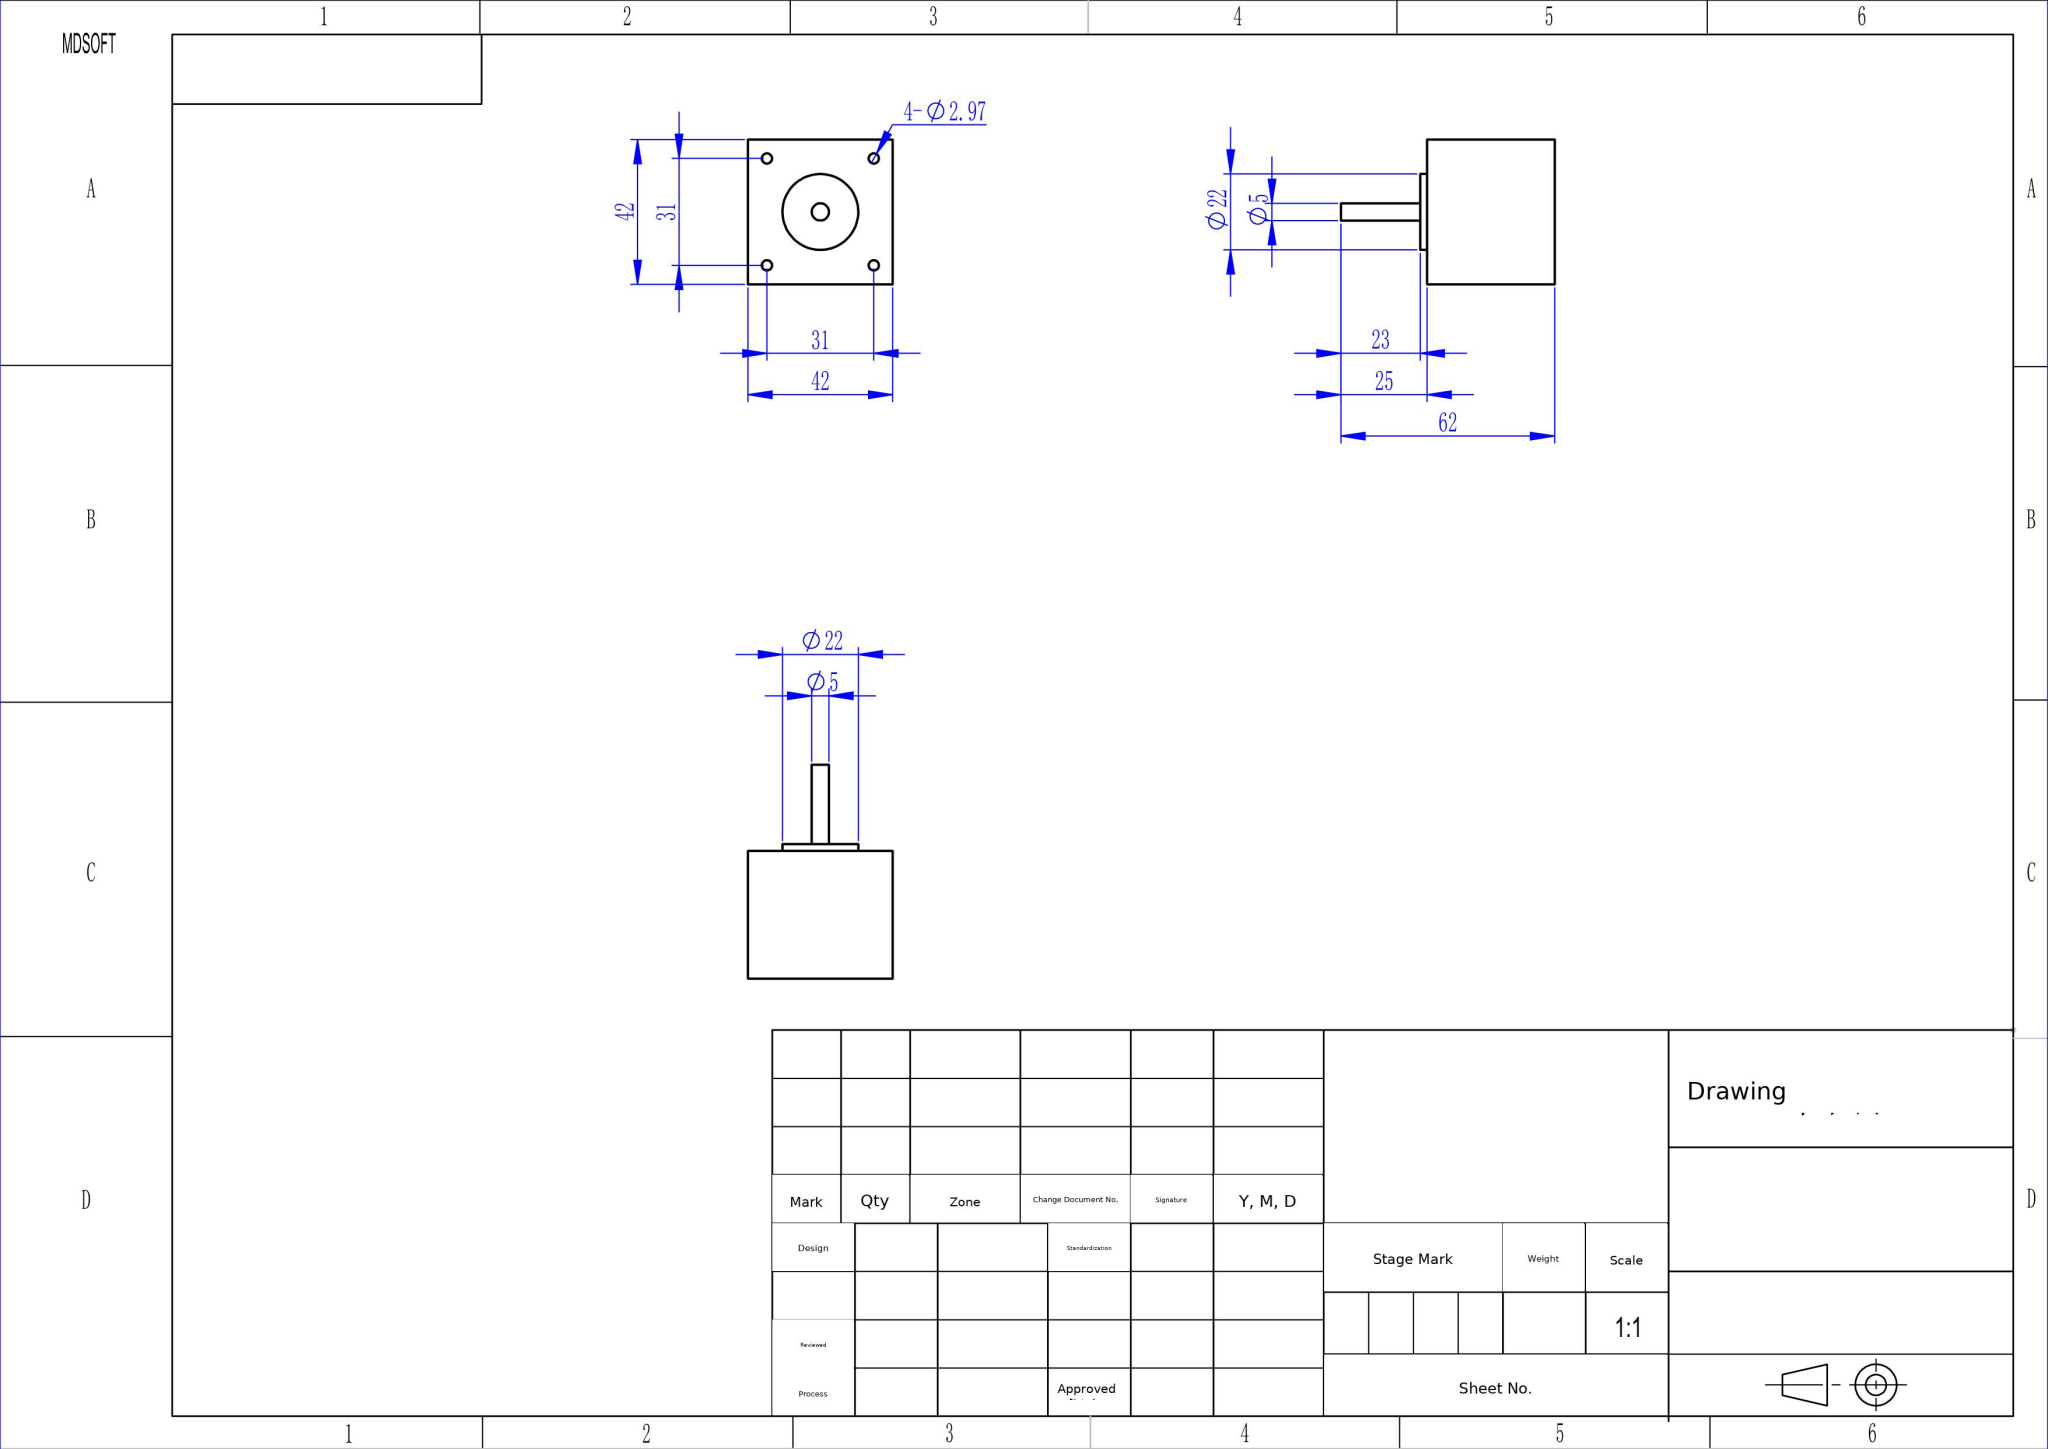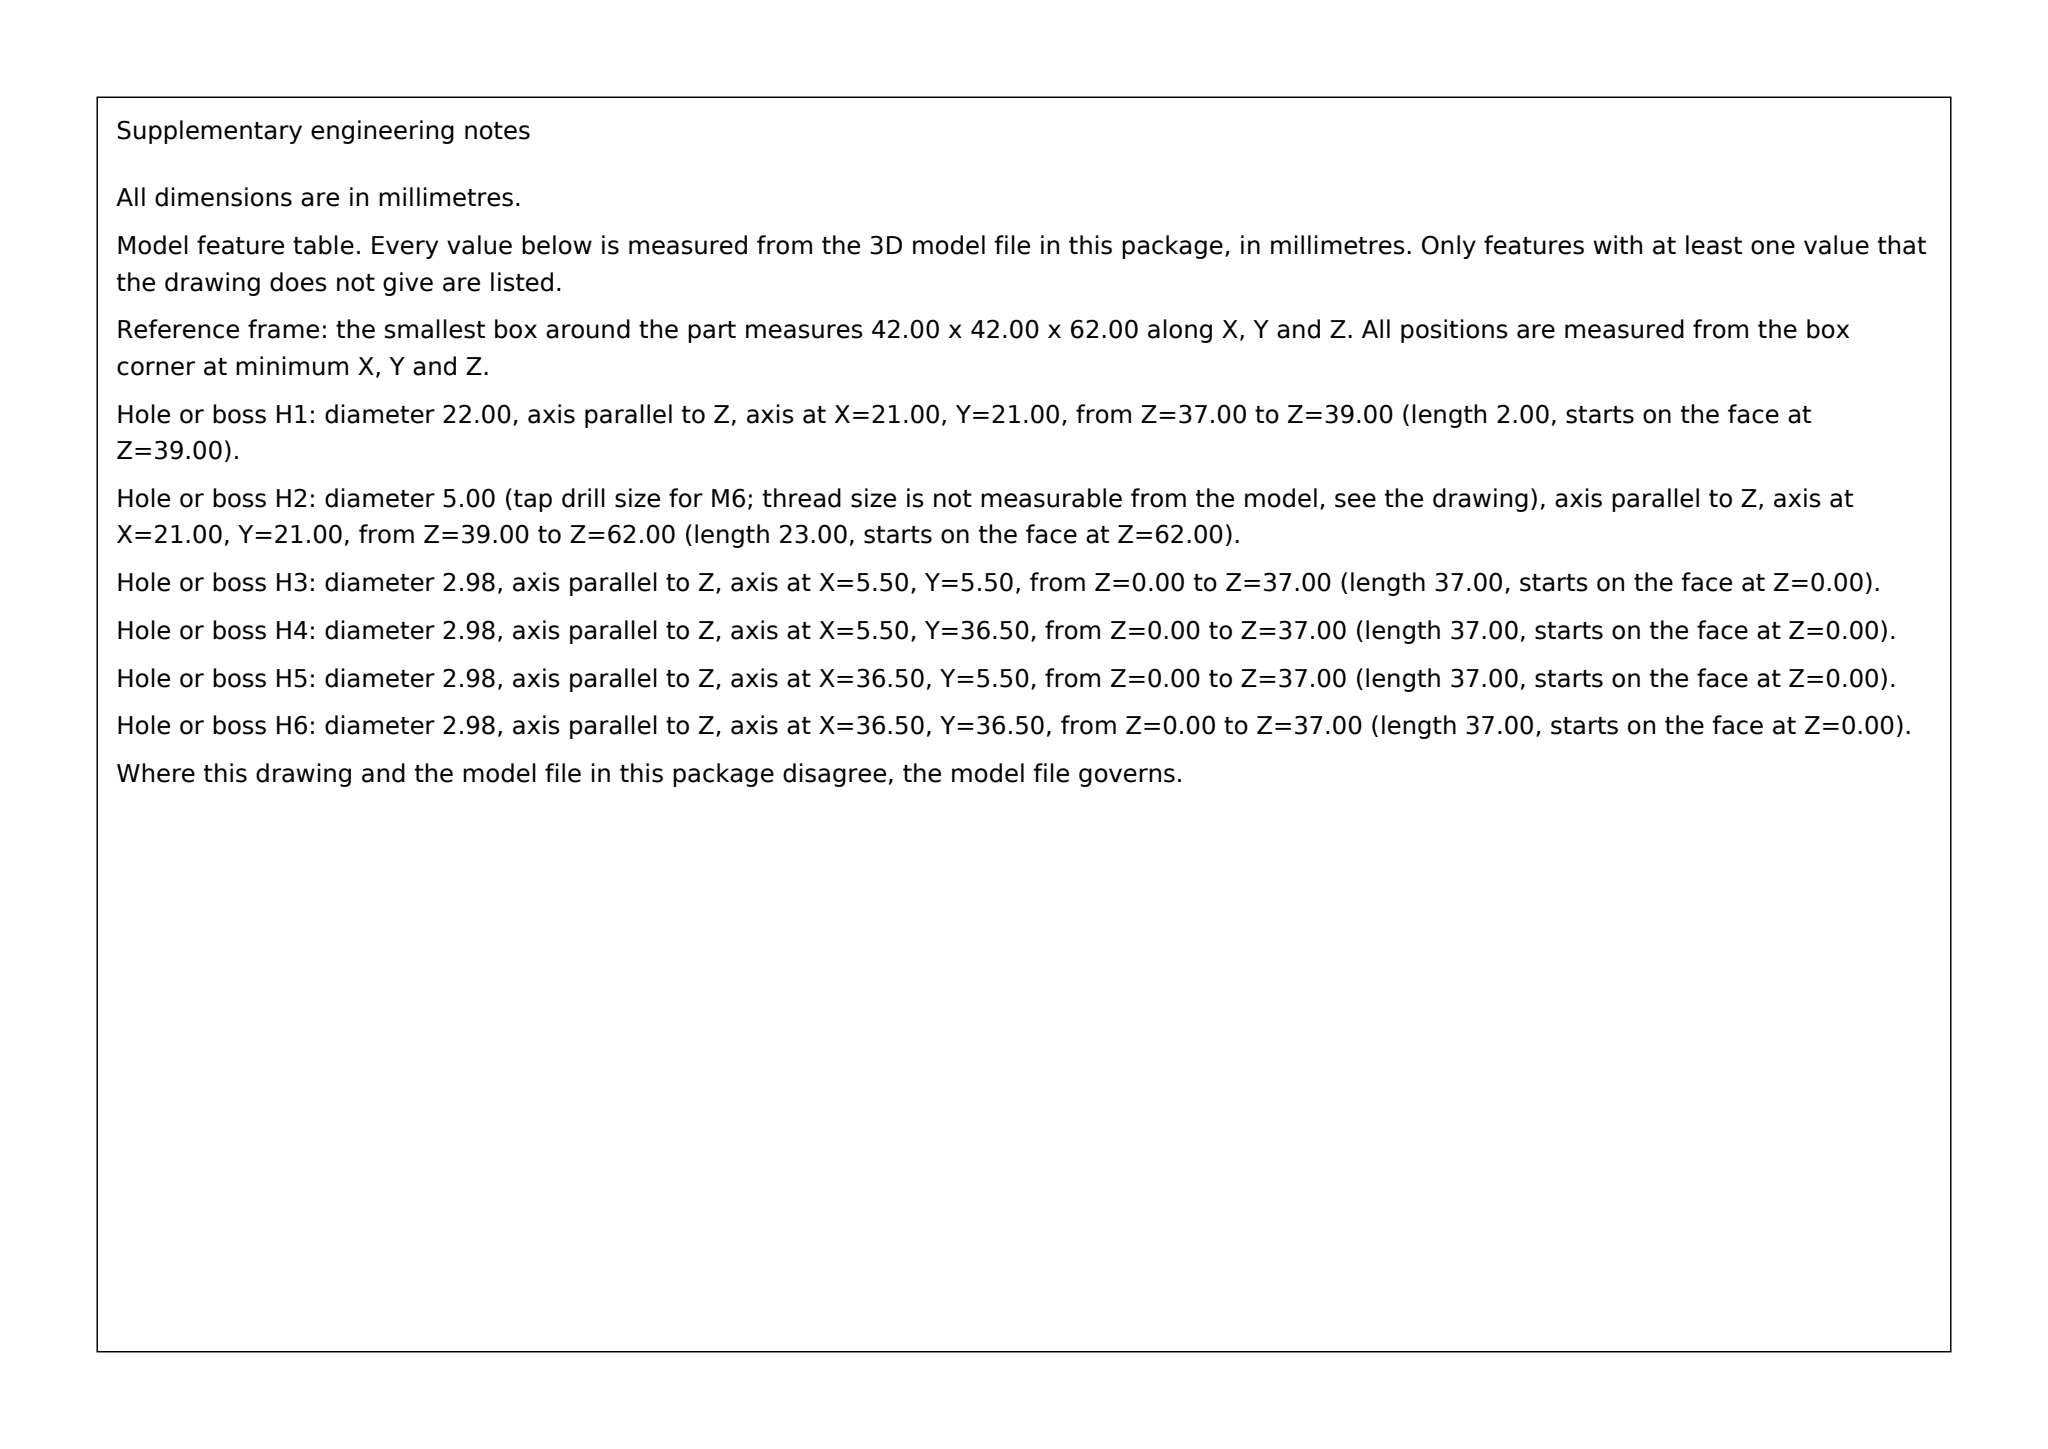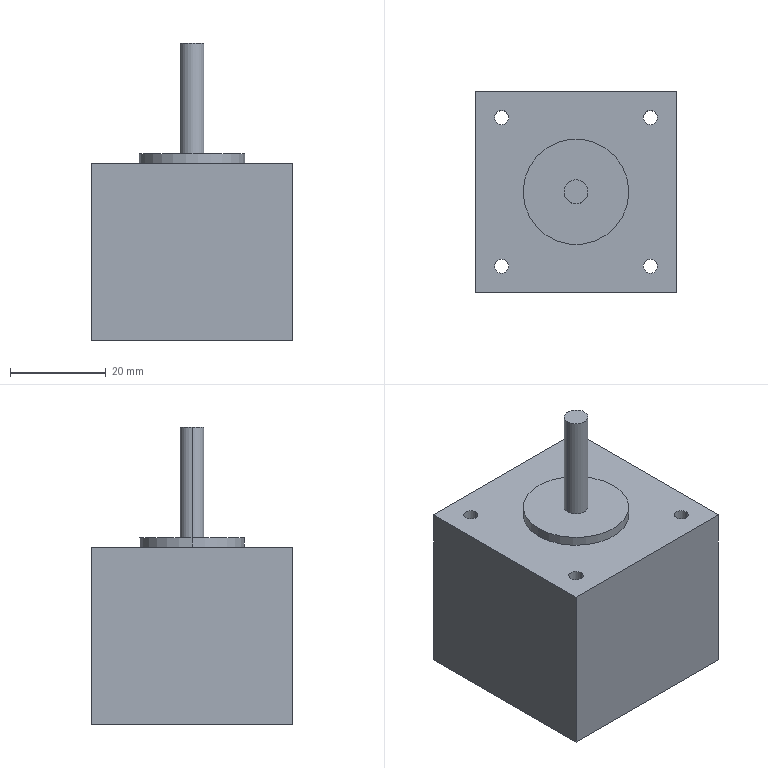Part | SolidWorks | mm | 1 solid | 20 faces | box 42 x 42 x 62 mm | volume 65453 mm3 | cylinder 12 | plane 8 | commonest cylinder face diameters 2.972 x8 5 x2 22 x2
build123d program:
from build123d import *

# Parameters (mm, degrees)
SKETCH1_W           = 42
SKETCH1_H           = 42
SKETCH1_R           = 1.486
BOSS_EXTRUDE1_DEPTH = 37
SKETCH3_3_R         = 2.5
BOSS_EXTRUDE2_DEPTH = 25
SKETCH3_3_2_R       = 11
SKETCH3_3_2_R_2     = 2.5
BOSS_EXTRUDE3_DEPTH = 2


with BuildPart() as part:
    # Sketch1 → Boss-Extrude1 (new body)
    with BuildSketch(Plane.XY):
        with Locations((-1.97, 1.739)):
            Rectangle(SKETCH1_W, SKETCH1_H)
        with Locations((-17.47, 17.239)):
            Circle(SKETCH1_R, mode=Mode.SUBTRACT)
        with Locations((13.53, 17.239)):
            Circle(SKETCH1_R, mode=Mode.SUBTRACT)
        with Locations((-17.47, -13.761)):
            Circle(SKETCH1_R, mode=Mode.SUBTRACT)
        with Locations((13.53, -13.761)):
            Circle(SKETCH1_R, mode=Mode.SUBTRACT)
    extrude(amount=BOSS_EXTRUDE1_DEPTH)



with BuildPart() as body_2:
    # Sketch3_3 → Boss-Extrude2 (new body)
    with BuildSketch(Plane.XY.offset(37)):
        with Locations((-1.97, 1.739)):
            Circle(SKETCH3_3_R)
    extrude(amount=BOSS_EXTRUDE2_DEPTH)


with BuildPart() as part_1:
    add(part.part)

    add(body_2.part)  # Boss-Extrude3 merges body 2
    # Sketch3_3 2 → Boss-Extrude3 (add)
    with BuildSketch(Plane.XY.offset(37)):
        with Locations((-1.97, 1.739)):
            Circle(SKETCH3_3_2_R)
        with Locations((-1.97, 1.739)):
            Circle(SKETCH3_3_2_R_2, mode=Mode.SUBTRACT)
    extrude(amount=BOSS_EXTRUDE3_DEPTH)


solid = part_1.part
STEP:
#1=CARTESIAN_POINT('',(0.5303,1.739,62.));
#2=VERTEX_POINT('',#1);
#3=CARTESIAN_POINT('',(-4.47,1.739,62.));
#4=VERTEX_POINT('',#3);
#5=CARTESIAN_POINT('',(-1.97,1.739,62.));
#6=DIRECTION('',(0.,0.,1.));
#7=DIRECTION('',(1.,0.,0.));
#8=AXIS2_PLACEMENT_3D('',#5,#6,#7);
#9=CIRCLE('',#8,2.5);
#10=EDGE_CURVE('',#2,#4,#9,.T.);
#11=ORIENTED_EDGE('',*,*,#10,.F.);
#12=CARTESIAN_POINT('',(0.5303,1.739,39.));
#13=VERTEX_POINT('',#12);
#14=CARTESIAN_POINT('',(0.5303,1.739,62.));
#15=DIRECTION('',(0.,0.,-1.));
#16=VECTOR('',#15,1000.);
#17=LINE('',#14,#16);
#18=EDGE_CURVE('',#2,#13,#17,.T.);
#19=ORIENTED_EDGE('',*,*,#18,.T.);
#20=CARTESIAN_POINT('',(-4.47,1.739,39.));
#21=VERTEX_POINT('',#20);
#22=CARTESIAN_POINT('',(-1.97,1.739,39.));
#23=DIRECTION('',(0.,0.,1.));
#24=DIRECTION('',(1.,0.,0.));
#25=AXIS2_PLACEMENT_3D('',#22,#23,#24);
#26=CIRCLE('',#25,2.5);
#27=EDGE_CURVE('',#13,#21,#26,.T.);
#28=ORIENTED_EDGE('',*,*,#27,.T.);
#29=CARTESIAN_POINT('',(-4.47,1.739,62.));
#30=DIRECTION('',(0.,0.,-1.));
#31=VECTOR('',#30,1000.);
#32=LINE('',#29,#31);
#33=EDGE_CURVE('',#4,#21,#32,.T.);
#34=ORIENTED_EDGE('',*,*,#33,.F.);
#35=EDGE_LOOP('',(#11,#19,#28,#34));
#36=FACE_OUTER_BOUND('',#35,.T.);
#37=CARTESIAN_POINT('',(-1.97,1.739,62.));
#38=DIRECTION('',(0.,0.,-1.));
#39=DIRECTION('',(-1.,0.,0.));
#40=AXIS2_PLACEMENT_3D('',#37,#38,#39);
#41=CYLINDRICAL_SURFACE('',#40,2.5);
#42=ADVANCED_FACE('',(#36),#41,.T.);
#43=CARTESIAN_POINT('',(9.03,1.739,39.));
#44=VERTEX_POINT('',#43);
#45=CARTESIAN_POINT('',(-12.97,1.739,39.));
#46=VERTEX_POINT('',#45);
#47=CARTESIAN_POINT('',(-1.97,1.739,39.));
#48=DIRECTION('',(0.,0.,1.));
#49=DIRECTION('',(1.,0.,0.));
#50=AXIS2_PLACEMENT_3D('',#47,#48,#49);
#51=CIRCLE('',#50,11.);
#52=EDGE_CURVE('',#44,#46,#51,.T.);
#53=ORIENTED_EDGE('',*,*,#52,.F.);
#54=CARTESIAN_POINT('',(9.03,1.739,37.));
#55=VERTEX_POINT('',#54);
#56=CARTESIAN_POINT('',(9.03,1.739,39.));
#57=DIRECTION('',(0.,0.,-1.));
#58=VECTOR('',#57,1000.);
#59=LINE('',#56,#58);
#60=EDGE_CURVE('',#44,#55,#59,.T.);
#61=ORIENTED_EDGE('',*,*,#60,.T.);
#62=CARTESIAN_POINT('',(-12.97,1.739,37.));
#63=VERTEX_POINT('',#62);
#64=CARTESIAN_POINT('',(-1.97,1.739,37.));
#65=DIRECTION('',(0.,0.,1.));
#66=DIRECTION('',(1.,0.,0.));
#67=AXIS2_PLACEMENT_3D('',#64,#65,#66);
#68=CIRCLE('',#67,11.);
#69=EDGE_CURVE('',#55,#63,#68,.T.);
#70=ORIENTED_EDGE('',*,*,#69,.T.);
#71=CARTESIAN_POINT('',(-12.97,1.739,39.));
#72=DIRECTION('',(0.,0.,-1.));
#73=VECTOR('',#72,1000.);
#74=LINE('',#71,#73);
#75=EDGE_CURVE('',#46,#63,#74,.T.);
#76=ORIENTED_EDGE('',*,*,#75,.F.);
#77=EDGE_LOOP('',(#53,#61,#70,#76));
#78=FACE_OUTER_BOUND('',#77,.T.);
#79=CARTESIAN_POINT('',(-1.97,1.739,39.));
#80=DIRECTION('',(0.,0.,-1.));
#81=DIRECTION('',(-1.,0.,0.));
#82=AXIS2_PLACEMENT_3D('',#79,#80,#81);
#83=CYLINDRICAL_SURFACE('',#82,11.);
#84=ADVANCED_FACE('',(#78),#83,.T.);
#85=CARTESIAN_POINT('',(12.044,-13.761,37.));
#86=VERTEX_POINT('',#85);
#87=CARTESIAN_POINT('',(15.016,-13.761,37.));
#88=VERTEX_POINT('',#87);
#89=CARTESIAN_POINT('',(13.53,-13.761,37.));
#90=DIRECTION('',(0.,0.,1.));
#91=DIRECTION('',(1.,0.,0.));
#92=AXIS2_PLACEMENT_3D('',#89,#90,#91);
#93=CIRCLE('',#92,1.486);
#94=EDGE_CURVE('',#86,#88,#93,.T.);
#95=ORIENTED_EDGE('',*,*,#94,.T.);
#96=CARTESIAN_POINT('',(15.016,-13.761,0.));
#97=VERTEX_POINT('',#96);
#98=CARTESIAN_POINT('',(15.016,-13.761,37.));
#99=DIRECTION('',(0.,0.,-1.));
#100=VECTOR('',#99,1000.);
#101=LINE('',#98,#100);
#102=EDGE_CURVE('',#88,#97,#101,.T.);
#103=ORIENTED_EDGE('',*,*,#102,.T.);
#104=CARTESIAN_POINT('',(12.044,-13.761,0.));
#105=VERTEX_POINT('',#104);
#106=CARTESIAN_POINT('',(13.53,-13.761,0.));
#107=DIRECTION('',(0.,0.,1.));
#108=DIRECTION('',(1.,0.,0.));
#109=AXIS2_PLACEMENT_3D('',#106,#107,#108);
#110=CIRCLE('',#109,1.486);
#111=EDGE_CURVE('',#105,#97,#110,.T.);
#112=ORIENTED_EDGE('',*,*,#111,.F.);
#113=CARTESIAN_POINT('',(12.044,-13.761,37.));
#114=DIRECTION('',(0.,0.,-1.));
#115=VECTOR('',#114,1000.);
#116=LINE('',#113,#115);
#117=EDGE_CURVE('',#86,#105,#116,.T.);
#118=ORIENTED_EDGE('',*,*,#117,.F.);
#119=EDGE_LOOP('',(#95,#103,#112,#118));
#120=FACE_OUTER_BOUND('',#119,.T.);
#121=CARTESIAN_POINT('',(13.53,-13.761,37.));
#122=DIRECTION('',(0.,0.,-1.));
#123=DIRECTION('',(-1.,0.,0.));
#124=AXIS2_PLACEMENT_3D('',#121,#122,#123);
#125=CYLINDRICAL_SURFACE('',#124,1.486);
#126=ADVANCED_FACE('',(#120),#125,.F.);
#127=CARTESIAN_POINT('',(-18.956,-13.761,37.));
#128=VERTEX_POINT('',#127);
#129=CARTESIAN_POINT('',(-15.984,-13.761,37.));
#130=VERTEX_POINT('',#129);
#131=CARTESIAN_POINT('',(-17.47,-13.761,37.));
#132=DIRECTION('',(0.,0.,1.));
#133=DIRECTION('',(1.,0.,0.));
#134=AXIS2_PLACEMENT_3D('',#131,#132,#133);
#135=CIRCLE('',#134,1.486);
#136=EDGE_CURVE('',#128,#130,#135,.T.);
#137=ORIENTED_EDGE('',*,*,#136,.T.);
#138=CARTESIAN_POINT('',(-15.984,-13.761,0.));
#139=VERTEX_POINT('',#138);
#140=CARTESIAN_POINT('',(-15.984,-13.761,37.));
#141=DIRECTION('',(0.,0.,-1.));
#142=VECTOR('',#141,1000.);
#143=LINE('',#140,#142);
#144=EDGE_CURVE('',#130,#139,#143,.T.);
#145=ORIENTED_EDGE('',*,*,#144,.T.);
#146=CARTESIAN_POINT('',(-18.956,-13.761,0.));
#147=VERTEX_POINT('',#146);
#148=CARTESIAN_POINT('',(-17.47,-13.761,0.));
#149=DIRECTION('',(0.,0.,1.));
#150=DIRECTION('',(1.,0.,0.));
#151=AXIS2_PLACEMENT_3D('',#148,#149,#150);
#152=CIRCLE('',#151,1.486);
#153=EDGE_CURVE('',#147,#139,#152,.T.);
#154=ORIENTED_EDGE('',*,*,#153,.F.);
#155=CARTESIAN_POINT('',(-18.956,-13.761,37.));
#156=DIRECTION('',(0.,0.,-1.));
#157=VECTOR('',#156,1000.);
#158=LINE('',#155,#157);
#159=EDGE_CURVE('',#128,#147,#158,.T.);
#160=ORIENTED_EDGE('',*,*,#159,.F.);
#161=EDGE_LOOP('',(#137,#145,#154,#160));
#162=FACE_OUTER_BOUND('',#161,.T.);
#163=CARTESIAN_POINT('',(-17.47,-13.761,37.));
#164=DIRECTION('',(0.,0.,-1.));
#165=DIRECTION('',(-1.,0.,0.));
#166=AXIS2_PLACEMENT_3D('',#163,#164,#165);
#167=CYLINDRICAL_SURFACE('',#166,1.486);
#168=ADVANCED_FACE('',(#162),#167,.F.);
#169=CARTESIAN_POINT('',(12.044,17.239,37.));
#170=VERTEX_POINT('',#169);
#171=CARTESIAN_POINT('',(15.016,17.239,37.));
#172=VERTEX_POINT('',#171);
#173=CARTESIAN_POINT('',(13.53,17.239,37.));
#174=DIRECTION('',(0.,0.,1.));
#175=DIRECTION('',(1.,0.,0.));
#176=AXIS2_PLACEMENT_3D('',#173,#174,#175);
#177=CIRCLE('',#176,1.486);
#178=EDGE_CURVE('',#170,#172,#177,.T.);
#179=ORIENTED_EDGE('',*,*,#178,.T.);
#180=CARTESIAN_POINT('',(15.016,17.239,0.));
#181=VERTEX_POINT('',#180);
#182=CARTESIAN_POINT('',(15.016,17.239,37.));
#183=DIRECTION('',(0.,0.,-1.));
#184=VECTOR('',#183,1000.);
#185=LINE('',#182,#184);
#186=EDGE_CURVE('',#172,#181,#185,.T.);
#187=ORIENTED_EDGE('',*,*,#186,.T.);
#188=CARTESIAN_POINT('',(12.044,17.239,0.));
#189=VERTEX_POINT('',#188);
#190=CARTESIAN_POINT('',(13.53,17.239,0.));
#191=DIRECTION('',(0.,0.,1.));
#192=DIRECTION('',(1.,0.,0.));
#193=AXIS2_PLACEMENT_3D('',#190,#191,#192);
#194=CIRCLE('',#193,1.486);
#195=EDGE_CURVE('',#189,#181,#194,.T.);
#196=ORIENTED_EDGE('',*,*,#195,.F.);
#197=CARTESIAN_POINT('',(12.044,17.239,37.));
#198=DIRECTION('',(0.,0.,-1.));
#199=VECTOR('',#198,1000.);
#200=LINE('',#197,#199);
#201=EDGE_CURVE('',#170,#189,#200,.T.);
#202=ORIENTED_EDGE('',*,*,#201,.F.);
#203=EDGE_LOOP('',(#179,#187,#196,#202));
#204=FACE_OUTER_BOUND('',#203,.T.);
#205=CARTESIAN_POINT('',(13.53,17.239,37.));
#206=DIRECTION('',(0.,0.,-1.));
#207=DIRECTION('',(-1.,0.,0.));
#208=AXIS2_PLACEMENT_3D('',#205,#206,#207);
#209=CYLINDRICAL_SURFACE('',#208,1.486);
#210=ADVANCED_FACE('',(#204),#209,.F.);
#211=CARTESIAN_POINT('',(-18.956,17.239,37.));
#212=VERTEX_POINT('',#211);
#213=CARTESIAN_POINT('',(-15.984,17.239,37.));
#214=VERTEX_POINT('',#213);
#215=CARTESIAN_POINT('',(-17.47,17.239,37.));
#216=DIRECTION('',(0.,0.,1.));
#217=DIRECTION('',(1.,0.,0.));
#218=AXIS2_PLACEMENT_3D('',#215,#216,#217);
#219=CIRCLE('',#218,1.486);
#220=EDGE_CURVE('',#212,#214,#219,.T.);
#221=ORIENTED_EDGE('',*,*,#220,.T.);
#222=CARTESIAN_POINT('',(-15.984,17.239,0.));
#223=VERTEX_POINT('',#222);
#224=CARTESIAN_POINT('',(-15.984,17.239,37.));
#225=DIRECTION('',(0.,0.,-1.));
#226=VECTOR('',#225,1000.);
#227=LINE('',#224,#226);
#228=EDGE_CURVE('',#214,#223,#227,.T.);
#229=ORIENTED_EDGE('',*,*,#228,.T.);
#230=CARTESIAN_POINT('',(-18.956,17.239,0.));
#231=VERTEX_POINT('',#230);
#232=CARTESIAN_POINT('',(-17.47,17.239,0.));
#233=DIRECTION('',(0.,0.,1.));
#234=DIRECTION('',(1.,0.,0.));
#235=AXIS2_PLACEMENT_3D('',#232,#233,#234);
#236=CIRCLE('',#235,1.486);
#237=EDGE_CURVE('',#231,#223,#236,.T.);
#238=ORIENTED_EDGE('',*,*,#237,.F.);
#239=CARTESIAN_POINT('',(-18.956,17.239,37.));
#240=DIRECTION('',(0.,0.,-1.));
#241=VECTOR('',#240,1000.);
#242=LINE('',#239,#241);
#243=EDGE_CURVE('',#212,#231,#242,.T.);
#244=ORIENTED_EDGE('',*,*,#243,.F.);
#245=EDGE_LOOP('',(#221,#229,#238,#244));
#246=FACE_OUTER_BOUND('',#245,.T.);
#247=CARTESIAN_POINT('',(-17.47,17.239,37.));
#248=DIRECTION('',(0.,0.,-1.));
#249=DIRECTION('',(-1.,0.,0.));
#250=AXIS2_PLACEMENT_3D('',#247,#248,#249);
#251=CYLINDRICAL_SURFACE('',#250,1.486);
#252=ADVANCED_FACE('',(#246),#251,.F.);
#253=CARTESIAN_POINT('',(-1.97,1.739,37.));
#254=DIRECTION('',(0.,0.,1.));
#255=DIRECTION('',(1.,0.,0.));
#256=AXIS2_PLACEMENT_3D('',#253,#254,#255);
#257=CIRCLE('',#256,11.);
#258=EDGE_CURVE('',#63,#55,#257,.T.);
#259=ORIENTED_EDGE('',*,*,#258,.F.);
#260=ORIENTED_EDGE('',*,*,#69,.F.);
#261=EDGE_LOOP('',(#259,#260));
#262=FACE_BOUND('',#261,.T.);
#263=ORIENTED_EDGE('',*,*,#136,.F.);
#264=CARTESIAN_POINT('',(-17.47,-13.761,37.));
#265=DIRECTION('',(0.,0.,1.));
#266=DIRECTION('',(1.,0.,0.));
#267=AXIS2_PLACEMENT_3D('',#264,#265,#266);
#268=CIRCLE('',#267,1.486);
#269=EDGE_CURVE('',#130,#128,#268,.T.);
#270=ORIENTED_EDGE('',*,*,#269,.F.);
#271=EDGE_LOOP('',(#263,#270));
#272=FACE_BOUND('',#271,.T.);
#273=ORIENTED_EDGE('',*,*,#220,.F.);
#274=CARTESIAN_POINT('',(-17.47,17.239,37.));
#275=DIRECTION('',(0.,0.,1.));
#276=DIRECTION('',(1.,0.,0.));
#277=AXIS2_PLACEMENT_3D('',#274,#275,#276);
#278=CIRCLE('',#277,1.486);
#279=EDGE_CURVE('',#214,#212,#278,.T.);
#280=ORIENTED_EDGE('',*,*,#279,.F.);
#281=EDGE_LOOP('',(#273,#280));
#282=FACE_BOUND('',#281,.T.);
#283=CARTESIAN_POINT('',(-22.97,22.739,37.));
#284=VERTEX_POINT('',#283);
#285=CARTESIAN_POINT('',(-22.97,-19.261,37.));
#286=VERTEX_POINT('',#285);
#287=CARTESIAN_POINT('',(-22.97,22.739,37.));
#288=DIRECTION('',(0.,-1.,0.));
#289=VECTOR('',#288,1000.);
#290=LINE('',#287,#289);
#291=EDGE_CURVE('',#284,#286,#290,.T.);
#292=ORIENTED_EDGE('',*,*,#291,.T.);
#293=CARTESIAN_POINT('',(19.03,-19.261,37.));
#294=VERTEX_POINT('',#293);
#295=CARTESIAN_POINT('',(-22.97,-19.261,37.));
#296=DIRECTION('',(1.,0.,0.));
#297=VECTOR('',#296,1000.);
#298=LINE('',#295,#297);
#299=EDGE_CURVE('',#286,#294,#298,.T.);
#300=ORIENTED_EDGE('',*,*,#299,.T.);
#301=CARTESIAN_POINT('',(19.03,22.739,37.));
#302=VERTEX_POINT('',#301);
#303=CARTESIAN_POINT('',(19.03,22.739,37.));
#304=DIRECTION('',(-0.,1.,0.));
#305=VECTOR('',#304,1000.);
#306=LINE('',#303,#305);
#307=EDGE_CURVE('',#294,#302,#306,.T.);
#308=ORIENTED_EDGE('',*,*,#307,.T.);
#309=CARTESIAN_POINT('',(-22.97,22.739,37.));
#310=DIRECTION('',(-1.,0.,0.));
#311=VECTOR('',#310,1000.);
#312=LINE('',#309,#311);
#313=EDGE_CURVE('',#302,#284,#312,.T.);
#314=ORIENTED_EDGE('',*,*,#313,.T.);
#315=EDGE_LOOP('',(#292,#300,#308,#314));
#316=FACE_OUTER_BOUND('',#315,.T.);
#317=ORIENTED_EDGE('',*,*,#178,.F.);
#318=CARTESIAN_POINT('',(13.53,17.239,37.));
#319=DIRECTION('',(0.,0.,1.));
#320=DIRECTION('',(1.,0.,0.));
#321=AXIS2_PLACEMENT_3D('',#318,#319,#320);
#322=CIRCLE('',#321,1.486);
#323=EDGE_CURVE('',#172,#170,#322,.T.);
#324=ORIENTED_EDGE('',*,*,#323,.F.);
#325=EDGE_LOOP('',(#317,#324));
#326=FACE_BOUND('',#325,.T.);
#327=ORIENTED_EDGE('',*,*,#94,.F.);
#328=CARTESIAN_POINT('',(13.53,-13.761,37.));
#329=DIRECTION('',(0.,0.,1.));
#330=DIRECTION('',(1.,0.,0.));
#331=AXIS2_PLACEMENT_3D('',#328,#329,#330);
#332=CIRCLE('',#331,1.486);
#333=EDGE_CURVE('',#88,#86,#332,.T.);
#334=ORIENTED_EDGE('',*,*,#333,.F.);
#335=EDGE_LOOP('',(#327,#334));
#336=FACE_BOUND('',#335,.T.);
#337=CARTESIAN_POINT('',(0.,0.,37.));
#338=DIRECTION('',(0.,0.,1.));
#339=DIRECTION('',(1.,0.,0.));
#340=AXIS2_PLACEMENT_3D('',#337,#338,#339);
#341=PLANE('',#340);
#342=ADVANCED_FACE('',(#262,#272,#282,#316,#326,#336),#341,.T.);
#343=CARTESIAN_POINT('',(-22.97,22.739,0.));
#344=VERTEX_POINT('',#343);
#345=CARTESIAN_POINT('',(-22.97,-19.261,0.));
#346=VERTEX_POINT('',#345);
#347=CARTESIAN_POINT('',(-22.97,22.739,0.));
#348=DIRECTION('',(0.,-1.,0.));
#349=VECTOR('',#348,1000.);
#350=LINE('',#347,#349);
#351=EDGE_CURVE('',#344,#346,#350,.T.);
#352=ORIENTED_EDGE('',*,*,#351,.F.);
#353=CARTESIAN_POINT('',(19.03,22.739,0.));
#354=VERTEX_POINT('',#353);
#355=CARTESIAN_POINT('',(-22.97,22.739,0.));
#356=DIRECTION('',(-1.,0.,0.));
#357=VECTOR('',#356,1000.);
#358=LINE('',#355,#357);
#359=EDGE_CURVE('',#354,#344,#358,.T.);
#360=ORIENTED_EDGE('',*,*,#359,.F.);
#361=CARTESIAN_POINT('',(19.03,-19.261,0.));
#362=VERTEX_POINT('',#361);
#363=CARTESIAN_POINT('',(19.03,22.739,0.));
#364=DIRECTION('',(-0.,1.,0.));
#365=VECTOR('',#364,1000.);
#366=LINE('',#363,#365);
#367=EDGE_CURVE('',#362,#354,#366,.T.);
#368=ORIENTED_EDGE('',*,*,#367,.F.);
#369=CARTESIAN_POINT('',(-22.97,-19.261,0.));
#370=DIRECTION('',(1.,0.,0.));
#371=VECTOR('',#370,1000.);
#372=LINE('',#369,#371);
#373=EDGE_CURVE('',#346,#362,#372,.T.);
#374=ORIENTED_EDGE('',*,*,#373,.F.);
#375=EDGE_LOOP('',(#352,#360,#368,#374));
#376=FACE_OUTER_BOUND('',#375,.T.);
#377=ORIENTED_EDGE('',*,*,#237,.T.);
#378=CARTESIAN_POINT('',(-17.47,17.239,0.));
#379=DIRECTION('',(0.,0.,1.));
#380=DIRECTION('',(1.,0.,0.));
#381=AXIS2_PLACEMENT_3D('',#378,#379,#380);
#382=CIRCLE('',#381,1.486);
#383=EDGE_CURVE('',#223,#231,#382,.T.);
#384=ORIENTED_EDGE('',*,*,#383,.T.);
#385=EDGE_LOOP('',(#377,#384));
#386=FACE_BOUND('',#385,.T.);
#387=ORIENTED_EDGE('',*,*,#195,.T.);
#388=CARTESIAN_POINT('',(13.53,17.239,0.));
#389=DIRECTION('',(0.,0.,1.));
#390=DIRECTION('',(1.,0.,0.));
#391=AXIS2_PLACEMENT_3D('',#388,#389,#390);
#392=CIRCLE('',#391,1.486);
#393=EDGE_CURVE('',#181,#189,#392,.T.);
#394=ORIENTED_EDGE('',*,*,#393,.T.);
#395=EDGE_LOOP('',(#387,#394));
#396=FACE_BOUND('',#395,.T.);
#397=ORIENTED_EDGE('',*,*,#153,.T.);
#398=CARTESIAN_POINT('',(-17.47,-13.761,0.));
#399=DIRECTION('',(0.,0.,1.));
#400=DIRECTION('',(1.,0.,0.));
#401=AXIS2_PLACEMENT_3D('',#398,#399,#400);
#402=CIRCLE('',#401,1.486);
#403=EDGE_CURVE('',#139,#147,#402,.T.);
#404=ORIENTED_EDGE('',*,*,#403,.T.);
#405=EDGE_LOOP('',(#397,#404));
#406=FACE_BOUND('',#405,.T.);
#407=ORIENTED_EDGE('',*,*,#111,.T.);
#408=CARTESIAN_POINT('',(13.53,-13.761,0.));
#409=DIRECTION('',(0.,0.,1.));
#410=DIRECTION('',(1.,0.,0.));
#411=AXIS2_PLACEMENT_3D('',#408,#409,#410);
#412=CIRCLE('',#411,1.486);
#413=EDGE_CURVE('',#97,#105,#412,.T.);
#414=ORIENTED_EDGE('',*,*,#413,.T.);
#415=EDGE_LOOP('',(#407,#414));
#416=FACE_BOUND('',#415,.T.);
#417=CARTESIAN_POINT('',(0.,0.,0.));
#418=DIRECTION('',(0.,0.,1.));
#419=DIRECTION('',(1.,0.,0.));
#420=AXIS2_PLACEMENT_3D('',#417,#418,#419);
#421=PLANE('',#420);
#422=ADVANCED_FACE('',(#376,#386,#396,#406,#416),#421,.F.);
#423=ORIENTED_EDGE('',*,*,#351,.T.);
#424=CARTESIAN_POINT('',(-22.97,-19.261,37.));
#425=DIRECTION('',(0.,0.,-1.));
#426=VECTOR('',#425,1000.);
#427=LINE('',#424,#426);
#428=EDGE_CURVE('',#286,#346,#427,.T.);
#429=ORIENTED_EDGE('',*,*,#428,.F.);
#430=ORIENTED_EDGE('',*,*,#291,.F.);
#431=CARTESIAN_POINT('',(-22.97,22.739,37.));
#432=DIRECTION('',(0.,0.,-1.));
#433=VECTOR('',#432,1000.);
#434=LINE('',#431,#433);
#435=EDGE_CURVE('',#284,#344,#434,.T.);
#436=ORIENTED_EDGE('',*,*,#435,.T.);
#437=EDGE_LOOP('',(#423,#429,#430,#436));
#438=FACE_OUTER_BOUND('',#437,.T.);
#439=CARTESIAN_POINT('',(-22.97,22.739,37.));
#440=DIRECTION('',(1.,0.,0.));
#441=DIRECTION('',(-0.,1.,0.));
#442=AXIS2_PLACEMENT_3D('',#439,#440,#441);
#443=PLANE('',#442);
#444=ADVANCED_FACE('',(#438),#443,.F.);
#445=ORIENTED_EDGE('',*,*,#373,.T.);
#446=CARTESIAN_POINT('',(19.03,-19.261,37.));
#447=DIRECTION('',(0.,0.,-1.));
#448=VECTOR('',#447,1000.);
#449=LINE('',#446,#448);
#450=EDGE_CURVE('',#294,#362,#449,.T.);
#451=ORIENTED_EDGE('',*,*,#450,.F.);
#452=ORIENTED_EDGE('',*,*,#299,.F.);
#453=ORIENTED_EDGE('',*,*,#428,.T.);
#454=EDGE_LOOP('',(#445,#451,#452,#453));
#455=FACE_OUTER_BOUND('',#454,.T.);
#456=CARTESIAN_POINT('',(-22.97,-19.261,37.));
#457=DIRECTION('',(0.,1.,0.));
#458=DIRECTION('',(0.,0.,1.));
#459=AXIS2_PLACEMENT_3D('',#456,#457,#458);
#460=PLANE('',#459);
#461=ADVANCED_FACE('',(#455),#460,.F.);
#462=ORIENTED_EDGE('',*,*,#367,.T.);
#463=CARTESIAN_POINT('',(19.03,22.739,37.));
#464=DIRECTION('',(0.,0.,-1.));
#465=VECTOR('',#464,1000.);
#466=LINE('',#463,#465);
#467=EDGE_CURVE('',#302,#354,#466,.T.);
#468=ORIENTED_EDGE('',*,*,#467,.F.);
#469=ORIENTED_EDGE('',*,*,#307,.F.);
#470=ORIENTED_EDGE('',*,*,#450,.T.);
#471=EDGE_LOOP('',(#462,#468,#469,#470));
#472=FACE_OUTER_BOUND('',#471,.T.);
#473=CARTESIAN_POINT('',(19.03,22.739,37.));
#474=DIRECTION('',(-1.,-0.,0.));
#475=DIRECTION('',(0.,-1.,0.));
#476=AXIS2_PLACEMENT_3D('',#473,#474,#475);
#477=PLANE('',#476);
#478=ADVANCED_FACE('',(#472),#477,.F.);
#479=ORIENTED_EDGE('',*,*,#359,.T.);
#480=ORIENTED_EDGE('',*,*,#435,.F.);
#481=ORIENTED_EDGE('',*,*,#313,.F.);
#482=ORIENTED_EDGE('',*,*,#467,.T.);
#483=EDGE_LOOP('',(#479,#480,#481,#482));
#484=FACE_OUTER_BOUND('',#483,.T.);
#485=CARTESIAN_POINT('',(-22.97,22.739,37.));
#486=DIRECTION('',(0.,-1.,0.));
#487=DIRECTION('',(0.,0.,-1.));
#488=AXIS2_PLACEMENT_3D('',#485,#486,#487);
#489=PLANE('',#488);
#490=ADVANCED_FACE('',(#484),#489,.F.);
#491=ORIENTED_EDGE('',*,*,#228,.F.);
#492=ORIENTED_EDGE('',*,*,#279,.T.);
#493=ORIENTED_EDGE('',*,*,#243,.T.);
#494=ORIENTED_EDGE('',*,*,#383,.F.);
#495=EDGE_LOOP('',(#491,#492,#493,#494));
#496=FACE_OUTER_BOUND('',#495,.T.);
#497=CARTESIAN_POINT('',(-17.47,17.239,37.));
#498=DIRECTION('',(0.,0.,-1.));
#499=DIRECTION('',(-1.,0.,0.));
#500=AXIS2_PLACEMENT_3D('',#497,#498,#499);
#501=CYLINDRICAL_SURFACE('',#500,1.486);
#502=ADVANCED_FACE('',(#496),#501,.F.);
#503=ORIENTED_EDGE('',*,*,#186,.F.);
#504=ORIENTED_EDGE('',*,*,#323,.T.);
#505=ORIENTED_EDGE('',*,*,#201,.T.);
#506=ORIENTED_EDGE('',*,*,#393,.F.);
#507=EDGE_LOOP('',(#503,#504,#505,#506));
#508=FACE_OUTER_BOUND('',#507,.T.);
#509=CARTESIAN_POINT('',(13.53,17.239,37.));
#510=DIRECTION('',(0.,0.,-1.));
#511=DIRECTION('',(-1.,0.,0.));
#512=AXIS2_PLACEMENT_3D('',#509,#510,#511);
#513=CYLINDRICAL_SURFACE('',#512,1.486);
#514=ADVANCED_FACE('',(#508),#513,.F.);
#515=ORIENTED_EDGE('',*,*,#144,.F.);
#516=ORIENTED_EDGE('',*,*,#269,.T.);
#517=ORIENTED_EDGE('',*,*,#159,.T.);
#518=ORIENTED_EDGE('',*,*,#403,.F.);
#519=EDGE_LOOP('',(#515,#516,#517,#518));
#520=FACE_OUTER_BOUND('',#519,.T.);
#521=CARTESIAN_POINT('',(-17.47,-13.761,37.));
#522=DIRECTION('',(0.,0.,-1.));
#523=DIRECTION('',(-1.,0.,0.));
#524=AXIS2_PLACEMENT_3D('',#521,#522,#523);
#525=CYLINDRICAL_SURFACE('',#524,1.486);
#526=ADVANCED_FACE('',(#520),#525,.F.);
#527=ORIENTED_EDGE('',*,*,#102,.F.);
#528=ORIENTED_EDGE('',*,*,#333,.T.);
#529=ORIENTED_EDGE('',*,*,#117,.T.);
#530=ORIENTED_EDGE('',*,*,#413,.F.);
#531=EDGE_LOOP('',(#527,#528,#529,#530));
#532=FACE_OUTER_BOUND('',#531,.T.);
#533=CARTESIAN_POINT('',(13.53,-13.761,37.));
#534=DIRECTION('',(0.,0.,-1.));
#535=DIRECTION('',(-1.,0.,0.));
#536=AXIS2_PLACEMENT_3D('',#533,#534,#535);
#537=CYLINDRICAL_SURFACE('',#536,1.486);
#538=ADVANCED_FACE('',(#532),#537,.F.);
#539=CARTESIAN_POINT('',(-1.97,1.739,39.));
#540=DIRECTION('',(0.,0.,1.));
#541=DIRECTION('',(1.,0.,0.));
#542=AXIS2_PLACEMENT_3D('',#539,#540,#541);
#543=CIRCLE('',#542,11.);
#544=EDGE_CURVE('',#46,#44,#543,.T.);
#545=ORIENTED_EDGE('',*,*,#544,.T.);
#546=ORIENTED_EDGE('',*,*,#52,.T.);
#547=EDGE_LOOP('',(#545,#546));
#548=FACE_OUTER_BOUND('',#547,.T.);
#549=CARTESIAN_POINT('',(-1.97,1.739,39.));
#550=DIRECTION('',(0.,0.,1.));
#551=DIRECTION('',(1.,0.,0.));
#552=AXIS2_PLACEMENT_3D('',#549,#550,#551);
#553=CIRCLE('',#552,2.5);
#554=EDGE_CURVE('',#21,#13,#553,.T.);
#555=ORIENTED_EDGE('',*,*,#554,.F.);
#556=ORIENTED_EDGE('',*,*,#27,.F.);
#557=EDGE_LOOP('',(#555,#556));
#558=FACE_BOUND('',#557,.T.);
#559=CARTESIAN_POINT('',(-1.97,1.739,39.));
#560=DIRECTION('',(0.,0.,1.));
#561=DIRECTION('',(1.,0.,0.));
#562=AXIS2_PLACEMENT_3D('',#559,#560,#561);
#563=PLANE('',#562);
#564=ADVANCED_FACE('',(#548,#558),#563,.T.);
#565=ORIENTED_EDGE('',*,*,#60,.F.);
#566=ORIENTED_EDGE('',*,*,#544,.F.);
#567=ORIENTED_EDGE('',*,*,#75,.T.);
#568=ORIENTED_EDGE('',*,*,#258,.T.);
#569=EDGE_LOOP('',(#565,#566,#567,#568));
#570=FACE_OUTER_BOUND('',#569,.T.);
#571=CARTESIAN_POINT('',(-1.97,1.739,39.));
#572=DIRECTION('',(0.,0.,-1.));
#573=DIRECTION('',(-1.,0.,0.));
#574=AXIS2_PLACEMENT_3D('',#571,#572,#573);
#575=CYLINDRICAL_SURFACE('',#574,11.);
#576=ADVANCED_FACE('',(#570),#575,.T.);
#577=ORIENTED_EDGE('',*,*,#18,.F.);
#578=CARTESIAN_POINT('',(-1.97,1.739,62.));
#579=DIRECTION('',(0.,0.,1.));
#580=DIRECTION('',(1.,0.,0.));
#581=AXIS2_PLACEMENT_3D('',#578,#579,#580);
#582=CIRCLE('',#581,2.5);
#583=EDGE_CURVE('',#4,#2,#582,.T.);
#584=ORIENTED_EDGE('',*,*,#583,.F.);
#585=ORIENTED_EDGE('',*,*,#33,.T.);
#586=ORIENTED_EDGE('',*,*,#554,.T.);
#587=EDGE_LOOP('',(#577,#584,#585,#586));
#588=FACE_OUTER_BOUND('',#587,.T.);
#589=CARTESIAN_POINT('',(-1.97,1.739,62.));
#590=DIRECTION('',(0.,0.,-1.));
#591=DIRECTION('',(-1.,0.,0.));
#592=AXIS2_PLACEMENT_3D('',#589,#590,#591);
#593=CYLINDRICAL_SURFACE('',#592,2.5);
#594=ADVANCED_FACE('',(#588),#593,.T.);
#595=ORIENTED_EDGE('',*,*,#583,.T.);
#596=ORIENTED_EDGE('',*,*,#10,.T.);
#597=EDGE_LOOP('',(#595,#596));
#598=FACE_OUTER_BOUND('',#597,.T.);
#599=CARTESIAN_POINT('',(-1.97,1.739,62.));
#600=DIRECTION('',(0.,0.,1.));
#601=DIRECTION('',(1.,0.,0.));
#602=AXIS2_PLACEMENT_3D('',#599,#600,#601);
#603=PLANE('',#602);
#604=ADVANCED_FACE('',(#598),#603,.T.);
#605=CLOSED_SHELL('',(#42,#84,#126,#168,#210,#252,#342,#422,#444,#461,#478,#490,#502,#514,#526,#538,#564,#576,#594,#604));
#606=MANIFOLD_SOLID_BREP('',#605);
#607=CARTESIAN_POINT('',(0.,0.,0.));
#608=DIRECTION('',(0.,0.,1.));
#609=DIRECTION('',(1.,0.,0.));
#610=AXIS2_PLACEMENT_3D('',#607,#608,#609);
#611=(LENGTH_UNIT()NAMED_UNIT(*)SI_UNIT(.MILLI.,.METRE.));
#612=UNCERTAINTY_MEASURE_WITH_UNIT(LENGTH_MEASURE(0.00001),#611,'','');
#613=(NAMED_UNIT(*)PLANE_ANGLE_UNIT()SI_UNIT($,.RADIAN.));
#614=(NAMED_UNIT(*)SI_UNIT($,.STERADIAN.)SOLID_ANGLE_UNIT());
#615=(GEOMETRIC_REPRESENTATION_CONTEXT(3)GLOBAL_UNCERTAINTY_ASSIGNED_CONTEXT((#612))GLOBAL_UNIT_ASSIGNED_CONTEXT((#611,#613,#614))REPRESENTATION_CONTEXT('',''));
#616=ADVANCED_BREP_SHAPE_REPRESENTATION('',(#606,#610),#615);